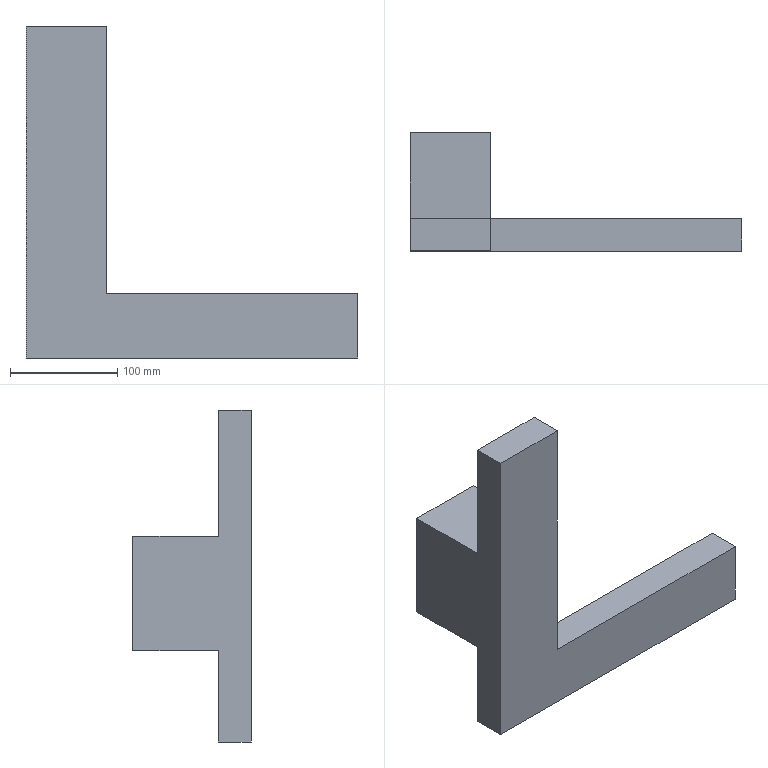Component | SolidWorks | MirrorPlate-2 | 1 solid | 19 faces | box 310 x 110.58 x 310 mm | volume 1628844 mm3 | plane 19
STEP:
#1=COLOUR_RGB('',0.7922,0.8196,0.9333);
#2=FILL_AREA_STYLE_COLOUR('',#1);
#3=FILL_AREA_STYLE('',(#2));
#4=SURFACE_STYLE_FILL_AREA(#3);
#5=SURFACE_SIDE_STYLE('',(#4));
#6=SURFACE_STYLE_USAGE(.BOTH.,#5);
#7=PRESENTATION_STYLE_ASSIGNMENT((#6));
#8=CARTESIAN_POINT('',(-6.62,1.886,11.6));
#9=VERTEX_POINT('',#8);
#10=CARTESIAN_POINT('',(-6.131,1.04,11.6));
#11=VERTEX_POINT('',#10);
#12=CARTESIAN_POINT('',(-6.131,1.04,11.6));
#13=DIRECTION('',(0.5,-0.866,-0.));
#14=VECTOR('',#13,39.37);
#15=LINE('',#12,#14);
#16=EDGE_CURVE('',#9,#11,#15,.T.);
#17=ORIENTED_EDGE('',*,*,#16,.F.);
#18=CARTESIAN_POINT('',(-6.62,1.886,7.781));
#19=VERTEX_POINT('',#18);
#20=CARTESIAN_POINT('',(-6.62,1.886,3.726));
#21=DIRECTION('',(0.,-0.,1.));
#22=VECTOR('',#21,39.37);
#23=LINE('',#20,#22);
#24=EDGE_CURVE('',#19,#9,#23,.T.);
#25=ORIENTED_EDGE('',*,*,#24,.F.);
#26=CARTESIAN_POINT('',(-6.131,1.04,7.781));
#27=VERTEX_POINT('',#26);
#28=CARTESIAN_POINT('',(-6.713,2.047,7.781));
#29=DIRECTION('',(-0.5,0.866,0.));
#30=VECTOR('',#29,39.37);
#31=LINE('',#28,#30);
#32=EDGE_CURVE('',#27,#19,#31,.T.);
#33=ORIENTED_EDGE('',*,*,#32,.F.);
#34=CARTESIAN_POINT('',(-6.131,1.04,3.726));
#35=DIRECTION('',(0.,-0.,1.));
#36=VECTOR('',#35,39.37);
#37=LINE('',#34,#36);
#38=EDGE_CURVE('',#27,#11,#37,.T.);
#39=ORIENTED_EDGE('',*,*,#38,.T.);
#40=EDGE_LOOP('',(#17,#25,#33,#39));
#41=FACE_OUTER_BOUND('',#40,.T.);
#42=CARTESIAN_POINT('',(-6.131,1.04,3.726));
#43=DIRECTION('',(0.866,0.5,0.));
#44=DIRECTION('',(0.5,-0.866,-0.));
#45=AXIS2_PLACEMENT_3D('',#42,#43,#44);
#46=PLANE('',#45);
#47=ADVANCED_FACE('',(#41),#46,.F.);
#48=CARTESIAN_POINT('',(-6.62,0.1934,11.6));
#49=VERTEX_POINT('',#48);
#50=CARTESIAN_POINT('',(-6.62,0.1934,11.6));
#51=DIRECTION('',(-0.5,-0.866,-0.));
#52=VECTOR('',#51,39.37);
#53=LINE('',#50,#52);
#54=EDGE_CURVE('',#11,#49,#53,.T.);
#55=ORIENTED_EDGE('',*,*,#54,.F.);
#56=ORIENTED_EDGE('',*,*,#38,.F.);
#57=CARTESIAN_POINT('',(-6.62,0.1934,7.781));
#58=VERTEX_POINT('',#57);
#59=CARTESIAN_POINT('',(-5.349,2.394,7.781));
#60=DIRECTION('',(0.5,0.866,0.));
#61=VECTOR('',#60,39.37);
#62=LINE('',#59,#61);
#63=EDGE_CURVE('',#58,#27,#62,.T.);
#64=ORIENTED_EDGE('',*,*,#63,.F.);
#65=CARTESIAN_POINT('',(-6.62,0.1934,3.726));
#66=DIRECTION('',(0.,-0.,1.));
#67=VECTOR('',#66,39.37);
#68=LINE('',#65,#67);
#69=EDGE_CURVE('',#58,#49,#68,.T.);
#70=ORIENTED_EDGE('',*,*,#69,.T.);
#71=EDGE_LOOP('',(#55,#56,#64,#70));
#72=FACE_OUTER_BOUND('',#71,.T.);
#73=CARTESIAN_POINT('',(-6.62,0.1934,3.726));
#74=DIRECTION('',(0.866,-0.5,-0.));
#75=DIRECTION('',(-0.5,-0.866,-0.));
#76=AXIS2_PLACEMENT_3D('',#73,#74,#75);
#77=PLANE('',#76);
#78=ADVANCED_FACE('',(#72),#77,.F.);
#79=CARTESIAN_POINT('',(-7.597,0.1934,11.6));
#80=VERTEX_POINT('',#79);
#81=CARTESIAN_POINT('',(-7.597,0.1934,11.6));
#82=DIRECTION('',(-1.,-0.,-0.));
#83=VECTOR('',#82,39.37);
#84=LINE('',#81,#83);
#85=EDGE_CURVE('',#49,#80,#84,.T.);
#86=ORIENTED_EDGE('',*,*,#85,.F.);
#87=ORIENTED_EDGE('',*,*,#69,.F.);
#88=CARTESIAN_POINT('',(-7.597,0.1934,7.781));
#89=VERTEX_POINT('',#88);
#90=CARTESIAN_POINT('',(-5.731,0.1934,7.781));
#91=DIRECTION('',(1.,0.,0.));
#92=VECTOR('',#91,39.37);
#93=LINE('',#90,#92);
#94=EDGE_CURVE('',#89,#58,#93,.T.);
#95=ORIENTED_EDGE('',*,*,#94,.F.);
#96=CARTESIAN_POINT('',(-7.597,0.1934,3.726));
#97=DIRECTION('',(0.,-0.,1.));
#98=VECTOR('',#97,39.37);
#99=LINE('',#96,#98);
#100=EDGE_CURVE('',#89,#80,#99,.T.);
#101=ORIENTED_EDGE('',*,*,#100,.T.);
#102=EDGE_LOOP('',(#86,#87,#95,#101));
#103=FACE_OUTER_BOUND('',#102,.T.);
#104=CARTESIAN_POINT('',(-7.597,0.1934,3.726));
#105=DIRECTION('',(0.,-1.,-0.));
#106=DIRECTION('',(-1.,-0.,-0.));
#107=AXIS2_PLACEMENT_3D('',#104,#105,#106);
#108=PLANE('',#107);
#109=ADVANCED_FACE('',(#103),#108,.F.);
#110=CARTESIAN_POINT('',(-8.086,1.04,11.6));
#111=VERTEX_POINT('',#110);
#112=CARTESIAN_POINT('',(-8.086,1.04,11.6));
#113=DIRECTION('',(-0.5,0.866,0.));
#114=VECTOR('',#113,39.37);
#115=LINE('',#112,#114);
#116=EDGE_CURVE('',#80,#111,#115,.T.);
#117=ORIENTED_EDGE('',*,*,#116,.F.);
#118=ORIENTED_EDGE('',*,*,#100,.F.);
#119=CARTESIAN_POINT('',(-8.086,1.04,7.781));
#120=VERTEX_POINT('',#119);
#121=CARTESIAN_POINT('',(-8.179,1.201,7.781));
#122=DIRECTION('',(0.5,-0.866,-0.));
#123=VECTOR('',#122,39.37);
#124=LINE('',#121,#123);
#125=EDGE_CURVE('',#120,#89,#124,.T.);
#126=ORIENTED_EDGE('',*,*,#125,.F.);
#127=CARTESIAN_POINT('',(-8.086,1.04,3.726));
#128=DIRECTION('',(0.,-0.,1.));
#129=VECTOR('',#128,39.37);
#130=LINE('',#127,#129);
#131=EDGE_CURVE('',#120,#111,#130,.T.);
#132=ORIENTED_EDGE('',*,*,#131,.T.);
#133=EDGE_LOOP('',(#117,#118,#126,#132));
#134=FACE_OUTER_BOUND('',#133,.T.);
#135=CARTESIAN_POINT('',(-8.086,1.04,3.726));
#136=DIRECTION('',(-0.866,-0.5,-0.));
#137=DIRECTION('',(-0.5,0.866,0.));
#138=AXIS2_PLACEMENT_3D('',#135,#136,#137);
#139=PLANE('',#138);
#140=ADVANCED_FACE('',(#134),#139,.F.);
#141=CARTESIAN_POINT('',(-7.597,1.886,11.6));
#142=VERTEX_POINT('',#141);
#143=CARTESIAN_POINT('',(-7.597,1.886,11.6));
#144=DIRECTION('',(0.5,0.866,0.));
#145=VECTOR('',#144,39.37);
#146=LINE('',#143,#145);
#147=EDGE_CURVE('',#111,#142,#146,.T.);
#148=ORIENTED_EDGE('',*,*,#147,.F.);
#149=ORIENTED_EDGE('',*,*,#131,.F.);
#150=CARTESIAN_POINT('',(-7.597,1.886,7.781));
#151=VERTEX_POINT('',#150);
#152=CARTESIAN_POINT('',(-6.815,3.241,7.781));
#153=DIRECTION('',(-0.5,-0.866,-0.));
#154=VECTOR('',#153,39.37);
#155=LINE('',#152,#154);
#156=EDGE_CURVE('',#151,#120,#155,.T.);
#157=ORIENTED_EDGE('',*,*,#156,.F.);
#158=CARTESIAN_POINT('',(-7.597,1.886,3.726));
#159=DIRECTION('',(0.,-0.,1.));
#160=VECTOR('',#159,39.37);
#161=LINE('',#158,#160);
#162=EDGE_CURVE('',#151,#142,#161,.T.);
#163=ORIENTED_EDGE('',*,*,#162,.T.);
#164=EDGE_LOOP('',(#148,#149,#157,#163));
#165=FACE_OUTER_BOUND('',#164,.T.);
#166=CARTESIAN_POINT('',(-7.597,1.886,3.726));
#167=DIRECTION('',(-0.866,0.5,0.));
#168=DIRECTION('',(0.5,0.866,0.));
#169=AXIS2_PLACEMENT_3D('',#166,#167,#168);
#170=PLANE('',#169);
#171=ADVANCED_FACE('',(#165),#170,.F.);
#172=CARTESIAN_POINT('',(-6.62,1.886,11.6));
#173=DIRECTION('',(1.,-0.,-0.));
#174=VECTOR('',#173,39.37);
#175=LINE('',#172,#174);
#176=EDGE_CURVE('',#142,#9,#175,.T.);
#177=ORIENTED_EDGE('',*,*,#176,.F.);
#178=ORIENTED_EDGE('',*,*,#162,.F.);
#179=CARTESIAN_POINT('',(-5.731,1.886,7.781));
#180=DIRECTION('',(-1.,0.,0.));
#181=VECTOR('',#180,39.37);
#182=LINE('',#179,#181);
#183=EDGE_CURVE('',#19,#151,#182,.T.);
#184=ORIENTED_EDGE('',*,*,#183,.F.);
#185=ORIENTED_EDGE('',*,*,#24,.T.);
#186=EDGE_LOOP('',(#177,#178,#184,#185));
#187=FACE_OUTER_BOUND('',#186,.T.);
#188=CARTESIAN_POINT('',(-6.62,1.886,3.726));
#189=DIRECTION('',(0.,1.,0.));
#190=DIRECTION('',(1.,-0.,-0.));
#191=AXIS2_PLACEMENT_3D('',#188,#189,#190);
#192=PLANE('',#191);
#193=ADVANCED_FACE('',(#187),#192,.F.);
#194=CARTESIAN_POINT('',(-5.731,-0.535,7.781));
#195=VERTEX_POINT('',#194);
#196=CARTESIAN_POINT('',(-8.683,-0.535,7.781));
#197=VERTEX_POINT('',#196);
#198=CARTESIAN_POINT('',(-5.731,-0.535,7.781));
#199=DIRECTION('',(-1.,0.,0.));
#200=VECTOR('',#199,39.37);
#201=LINE('',#198,#200);
#202=EDGE_CURVE('',#195,#197,#201,.T.);
#203=ORIENTED_EDGE('',*,*,#202,.F.);
#204=CARTESIAN_POINT('',(-5.731,-0.535,6.797));
#205=VERTEX_POINT('',#204);
#206=CARTESIAN_POINT('',(-5.731,-0.535,16.64));
#207=DIRECTION('',(0.,0.,-1.));
#208=VECTOR('',#207,39.37);
#209=LINE('',#206,#208);
#210=EDGE_CURVE('',#195,#205,#209,.T.);
#211=ORIENTED_EDGE('',*,*,#210,.T.);
#212=CARTESIAN_POINT('',(3.521,-0.535,6.797));
#213=VERTEX_POINT('',#212);
#214=CARTESIAN_POINT('',(-8.683,-0.535,6.797));
#215=DIRECTION('',(1.,-0.,-0.));
#216=VECTOR('',#215,39.37);
#217=LINE('',#214,#216);
#218=EDGE_CURVE('',#205,#213,#217,.T.);
#219=ORIENTED_EDGE('',*,*,#218,.T.);
#220=CARTESIAN_POINT('',(3.521,-0.535,4.435));
#221=VERTEX_POINT('',#220);
#222=CARTESIAN_POINT('',(3.521,-0.535,6.797));
#223=DIRECTION('',(0.,-0.,1.));
#224=VECTOR('',#223,39.37);
#225=LINE('',#222,#224);
#226=EDGE_CURVE('',#221,#213,#225,.T.);
#227=ORIENTED_EDGE('',*,*,#226,.F.);
#228=CARTESIAN_POINT('',(-8.683,-0.535,4.435));
#229=VERTEX_POINT('',#228);
#230=CARTESIAN_POINT('',(-8.683,-0.535,4.435));
#231=DIRECTION('',(1.,-0.,-0.));
#232=VECTOR('',#231,39.37);
#233=LINE('',#230,#232);
#234=EDGE_CURVE('',#229,#221,#233,.T.);
#235=ORIENTED_EDGE('',*,*,#234,.F.);
#236=CARTESIAN_POINT('',(-8.683,-0.535,6.797));
#237=DIRECTION('',(0.,-0.,1.));
#238=VECTOR('',#237,39.37);
#239=LINE('',#236,#238);
#240=EDGE_CURVE('',#229,#197,#239,.T.);
#241=ORIENTED_EDGE('',*,*,#240,.T.);
#242=EDGE_LOOP('',(#203,#211,#219,#227,#235,#241));
#243=FACE_OUTER_BOUND('',#242,.T.);
#244=CARTESIAN_POINT('',(-8.683,-0.535,6.797));
#245=DIRECTION('',(-0.,-1.,-0.));
#246=DIRECTION('',(1.,-0.,-0.));
#247=AXIS2_PLACEMENT_3D('',#244,#245,#246);
#248=PLANE('',#247);
#249=ADVANCED_FACE('',(#243),#248,.F.);
#250=CARTESIAN_POINT('',(-8.683,-0.535,11.994));
#251=VERTEX_POINT('',#250);
#252=CARTESIAN_POINT('',(-5.731,-0.535,11.994));
#253=VERTEX_POINT('',#252);
#254=CARTESIAN_POINT('',(-5.731,-0.535,11.994));
#255=DIRECTION('',(1.,-0.,-0.));
#256=VECTOR('',#255,39.37);
#257=LINE('',#254,#256);
#258=EDGE_CURVE('',#251,#253,#257,.T.);
#259=ORIENTED_EDGE('',*,*,#258,.F.);
#260=CARTESIAN_POINT('',(-8.683,-0.535,16.64));
#261=VERTEX_POINT('',#260);
#262=CARTESIAN_POINT('',(-8.683,-0.535,6.797));
#263=DIRECTION('',(0.,-0.,1.));
#264=VECTOR('',#263,39.37);
#265=LINE('',#262,#264);
#266=EDGE_CURVE('',#251,#261,#265,.T.);
#267=ORIENTED_EDGE('',*,*,#266,.T.);
#268=CARTESIAN_POINT('',(-5.731,-0.535,16.64));
#269=VERTEX_POINT('',#268);
#270=CARTESIAN_POINT('',(-5.731,-0.535,16.64));
#271=DIRECTION('',(1.,-0.,-0.));
#272=VECTOR('',#271,39.37);
#273=LINE('',#270,#272);
#274=EDGE_CURVE('',#261,#269,#273,.T.);
#275=ORIENTED_EDGE('',*,*,#274,.T.);
#276=CARTESIAN_POINT('',(-5.731,-0.535,16.64));
#277=DIRECTION('',(0.,0.,-1.));
#278=VECTOR('',#277,39.37);
#279=LINE('',#276,#278);
#280=EDGE_CURVE('',#269,#253,#279,.T.);
#281=ORIENTED_EDGE('',*,*,#280,.T.);
#282=EDGE_LOOP('',(#259,#267,#275,#281));
#283=FACE_OUTER_BOUND('',#282,.T.);
#284=CARTESIAN_POINT('',(-8.683,-0.535,6.797));
#285=DIRECTION('',(-0.,-1.,-0.));
#286=DIRECTION('',(1.,-0.,-0.));
#287=AXIS2_PLACEMENT_3D('',#284,#285,#286);
#288=PLANE('',#287);
#289=ADVANCED_FACE('',(#283),#288,.F.);
#290=CARTESIAN_POINT('',(-5.731,-1.739,6.797));
#291=VERTEX_POINT('',#290);
#292=CARTESIAN_POINT('',(-5.731,-0.535,6.797));
#293=DIRECTION('',(-0.,-1.,-0.));
#294=VECTOR('',#293,39.37);
#295=LINE('',#292,#294);
#296=EDGE_CURVE('',#205,#291,#295,.T.);
#297=ORIENTED_EDGE('',*,*,#296,.T.);
#298=CARTESIAN_POINT('',(3.521,-1.739,6.797));
#299=VERTEX_POINT('',#298);
#300=CARTESIAN_POINT('',(-8.683,-1.739,6.797));
#301=DIRECTION('',(1.,-0.,-0.));
#302=VECTOR('',#301,39.37);
#303=LINE('',#300,#302);
#304=EDGE_CURVE('',#291,#299,#303,.T.);
#305=ORIENTED_EDGE('',*,*,#304,.T.);
#306=CARTESIAN_POINT('',(3.521,-0.535,6.797));
#307=DIRECTION('',(-0.,-1.,-0.));
#308=VECTOR('',#307,39.37);
#309=LINE('',#306,#308);
#310=EDGE_CURVE('',#213,#299,#309,.T.);
#311=ORIENTED_EDGE('',*,*,#310,.F.);
#312=ORIENTED_EDGE('',*,*,#218,.F.);
#313=EDGE_LOOP('',(#297,#305,#311,#312));
#314=FACE_OUTER_BOUND('',#313,.T.);
#315=CARTESIAN_POINT('',(-8.683,-0.535,6.797));
#316=DIRECTION('',(0.,0.,-1.));
#317=DIRECTION('',(1.,-0.,-0.));
#318=AXIS2_PLACEMENT_3D('',#315,#316,#317);
#319=PLANE('',#318);
#320=ADVANCED_FACE('',(#314),#319,.F.);
#321=CARTESIAN_POINT('',(3.521,-1.739,4.435));
#322=VERTEX_POINT('',#321);
#323=CARTESIAN_POINT('',(3.521,-1.739,6.797));
#324=DIRECTION('',(0.,0.,-1.));
#325=VECTOR('',#324,39.37);
#326=LINE('',#323,#325);
#327=EDGE_CURVE('',#299,#322,#326,.T.);
#328=ORIENTED_EDGE('',*,*,#327,.F.);
#329=ORIENTED_EDGE('',*,*,#304,.F.);
#330=CARTESIAN_POINT('',(-5.731,-1.739,16.64));
#331=VERTEX_POINT('',#330);
#332=CARTESIAN_POINT('',(-5.731,-1.739,16.64));
#333=DIRECTION('',(0.,0.,-1.));
#334=VECTOR('',#333,39.37);
#335=LINE('',#332,#334);
#336=EDGE_CURVE('',#331,#291,#335,.T.);
#337=ORIENTED_EDGE('',*,*,#336,.F.);
#338=CARTESIAN_POINT('',(-8.683,-1.739,16.64));
#339=VERTEX_POINT('',#338);
#340=CARTESIAN_POINT('',(-5.731,-1.739,16.64));
#341=DIRECTION('',(-1.,0.,0.));
#342=VECTOR('',#341,39.37);
#343=LINE('',#340,#342);
#344=EDGE_CURVE('',#331,#339,#343,.T.);
#345=ORIENTED_EDGE('',*,*,#344,.T.);
#346=CARTESIAN_POINT('',(-8.683,-1.739,4.435));
#347=VERTEX_POINT('',#346);
#348=CARTESIAN_POINT('',(-8.683,-1.739,6.797));
#349=DIRECTION('',(0.,0.,-1.));
#350=VECTOR('',#349,39.37);
#351=LINE('',#348,#350);
#352=EDGE_CURVE('',#339,#347,#351,.T.);
#353=ORIENTED_EDGE('',*,*,#352,.T.);
#354=CARTESIAN_POINT('',(-8.683,-1.739,4.435));
#355=DIRECTION('',(1.,-0.,-0.));
#356=VECTOR('',#355,39.37);
#357=LINE('',#354,#356);
#358=EDGE_CURVE('',#347,#322,#357,.T.);
#359=ORIENTED_EDGE('',*,*,#358,.T.);
#360=EDGE_LOOP('',(#328,#329,#337,#345,#353,#359));
#361=FACE_OUTER_BOUND('',#360,.T.);
#362=CARTESIAN_POINT('',(-8.683,-1.739,6.797));
#363=DIRECTION('',(0.,1.,0.));
#364=DIRECTION('',(-1.,0.,0.));
#365=AXIS2_PLACEMENT_3D('',#362,#363,#364);
#366=PLANE('',#365);
#367=ADVANCED_FACE('',(#361),#366,.F.);
#368=CARTESIAN_POINT('',(3.521,-0.535,4.435));
#369=DIRECTION('',(0.,1.,0.));
#370=VECTOR('',#369,39.37);
#371=LINE('',#368,#370);
#372=EDGE_CURVE('',#322,#221,#371,.T.);
#373=ORIENTED_EDGE('',*,*,#372,.F.);
#374=ORIENTED_EDGE('',*,*,#358,.F.);
#375=CARTESIAN_POINT('',(-8.683,-0.535,4.435));
#376=DIRECTION('',(0.,1.,0.));
#377=VECTOR('',#376,39.37);
#378=LINE('',#375,#377);
#379=EDGE_CURVE('',#347,#229,#378,.T.);
#380=ORIENTED_EDGE('',*,*,#379,.T.);
#381=ORIENTED_EDGE('',*,*,#234,.T.);
#382=EDGE_LOOP('',(#373,#374,#380,#381));
#383=FACE_OUTER_BOUND('',#382,.T.);
#384=CARTESIAN_POINT('',(-8.683,-0.535,4.435));
#385=DIRECTION('',(0.,-0.,1.));
#386=DIRECTION('',(-1.,0.,0.));
#387=AXIS2_PLACEMENT_3D('',#384,#385,#386);
#388=PLANE('',#387);
#389=ADVANCED_FACE('',(#383),#388,.F.);
#390=ORIENTED_EDGE('',*,*,#266,.F.);
#391=CARTESIAN_POINT('',(-8.683,2.615,11.994));
#392=VERTEX_POINT('',#391);
#393=CARTESIAN_POINT('',(-8.683,2.615,11.994));
#394=DIRECTION('',(-0.,-1.,-0.));
#395=VECTOR('',#394,39.37);
#396=LINE('',#393,#395);
#397=EDGE_CURVE('',#392,#251,#396,.T.);
#398=ORIENTED_EDGE('',*,*,#397,.F.);
#399=CARTESIAN_POINT('',(-8.683,2.615,7.781));
#400=VERTEX_POINT('',#399);
#401=CARTESIAN_POINT('',(-8.683,2.615,7.781));
#402=DIRECTION('',(0.,-0.,1.));
#403=VECTOR('',#402,39.37);
#404=LINE('',#401,#403);
#405=EDGE_CURVE('',#400,#392,#404,.T.);
#406=ORIENTED_EDGE('',*,*,#405,.F.);
#407=CARTESIAN_POINT('',(-8.683,2.615,7.781));
#408=DIRECTION('',(-0.,-1.,-0.));
#409=VECTOR('',#408,39.37);
#410=LINE('',#407,#409);
#411=EDGE_CURVE('',#400,#197,#410,.T.);
#412=ORIENTED_EDGE('',*,*,#411,.T.);
#413=ORIENTED_EDGE('',*,*,#240,.F.);
#414=ORIENTED_EDGE('',*,*,#379,.F.);
#415=ORIENTED_EDGE('',*,*,#352,.F.);
#416=CARTESIAN_POINT('',(-8.683,-0.535,16.64));
#417=DIRECTION('',(0.,1.,0.));
#418=VECTOR('',#417,39.37);
#419=LINE('',#416,#418);
#420=EDGE_CURVE('',#339,#261,#419,.T.);
#421=ORIENTED_EDGE('',*,*,#420,.T.);
#422=EDGE_LOOP('',(#390,#398,#406,#412,#413,#414,#415,#421));
#423=FACE_OUTER_BOUND('',#422,.T.);
#424=CARTESIAN_POINT('',(-8.683,-0.,-0.1851));
#425=DIRECTION('',(-1.,0.,0.));
#426=DIRECTION('',(0.,0.,-1.));
#427=AXIS2_PLACEMENT_3D('',#424,#425,#426);
#428=PLANE('',#427);
#429=ADVANCED_FACE('',(#423),#428,.T.);
#430=ORIENTED_EDGE('',*,*,#310,.T.);
#431=ORIENTED_EDGE('',*,*,#327,.T.);
#432=ORIENTED_EDGE('',*,*,#372,.T.);
#433=ORIENTED_EDGE('',*,*,#226,.T.);
#434=EDGE_LOOP('',(#430,#431,#432,#433));
#435=FACE_OUTER_BOUND('',#434,.T.);
#436=CARTESIAN_POINT('',(3.521,-0.,-0.1851));
#437=DIRECTION('',(-1.,0.,0.));
#438=DIRECTION('',(0.,0.,-1.));
#439=AXIS2_PLACEMENT_3D('',#436,#437,#438);
#440=PLANE('',#439);
#441=ADVANCED_FACE('',(#435),#440,.F.);
#442=CARTESIAN_POINT('',(-5.731,2.615,11.994));
#443=VERTEX_POINT('',#442);
#444=CARTESIAN_POINT('',(-5.731,2.615,11.994));
#445=DIRECTION('',(-0.,-1.,-0.));
#446=VECTOR('',#445,39.37);
#447=LINE('',#444,#446);
#448=EDGE_CURVE('',#443,#253,#447,.T.);
#449=ORIENTED_EDGE('',*,*,#448,.T.);
#450=ORIENTED_EDGE('',*,*,#280,.F.);
#451=CARTESIAN_POINT('',(-5.731,-0.535,16.64));
#452=DIRECTION('',(-0.,-1.,-0.));
#453=VECTOR('',#452,39.37);
#454=LINE('',#451,#453);
#455=EDGE_CURVE('',#269,#331,#454,.T.);
#456=ORIENTED_EDGE('',*,*,#455,.T.);
#457=ORIENTED_EDGE('',*,*,#336,.T.);
#458=ORIENTED_EDGE('',*,*,#296,.F.);
#459=ORIENTED_EDGE('',*,*,#210,.F.);
#460=CARTESIAN_POINT('',(-5.731,2.615,7.781));
#461=VERTEX_POINT('',#460);
#462=CARTESIAN_POINT('',(-5.731,2.615,7.781));
#463=DIRECTION('',(-0.,-1.,-0.));
#464=VECTOR('',#463,39.37);
#465=LINE('',#462,#464);
#466=EDGE_CURVE('',#461,#195,#465,.T.);
#467=ORIENTED_EDGE('',*,*,#466,.F.);
#468=CARTESIAN_POINT('',(-5.731,2.615,7.781));
#469=DIRECTION('',(0.,0.,-1.));
#470=VECTOR('',#469,39.37);
#471=LINE('',#468,#470);
#472=EDGE_CURVE('',#443,#461,#471,.T.);
#473=ORIENTED_EDGE('',*,*,#472,.F.);
#474=EDGE_LOOP('',(#449,#450,#456,#457,#458,#459,#467,#473));
#475=FACE_OUTER_BOUND('',#474,.T.);
#476=CARTESIAN_POINT('',(-5.731,-0.535,16.64));
#477=DIRECTION('',(-1.,0.,0.));
#478=DIRECTION('',(0.,0.,-1.));
#479=AXIS2_PLACEMENT_3D('',#476,#477,#478);
#480=PLANE('',#479);
#481=ADVANCED_FACE('',(#475),#480,.F.);
#482=ORIENTED_EDGE('',*,*,#455,.F.);
#483=ORIENTED_EDGE('',*,*,#274,.F.);
#484=ORIENTED_EDGE('',*,*,#420,.F.);
#485=ORIENTED_EDGE('',*,*,#344,.F.);
#486=EDGE_LOOP('',(#482,#483,#484,#485));
#487=FACE_OUTER_BOUND('',#486,.T.);
#488=CARTESIAN_POINT('',(3.521,-0.,16.64));
#489=DIRECTION('',(0.,-0.,1.));
#490=DIRECTION('',(-1.,0.,0.));
#491=AXIS2_PLACEMENT_3D('',#488,#489,#490);
#492=PLANE('',#491);
#493=ADVANCED_FACE('',(#487),#492,.T.);
#494=ORIENTED_EDGE('',*,*,#63,.T.);
#495=ORIENTED_EDGE('',*,*,#32,.T.);
#496=ORIENTED_EDGE('',*,*,#183,.T.);
#497=ORIENTED_EDGE('',*,*,#156,.T.);
#498=ORIENTED_EDGE('',*,*,#125,.T.);
#499=ORIENTED_EDGE('',*,*,#94,.T.);
#500=EDGE_LOOP('',(#494,#495,#496,#497,#498,#499));
#501=FACE_BOUND('',#500,.T.);
#502=ORIENTED_EDGE('',*,*,#466,.T.);
#503=ORIENTED_EDGE('',*,*,#202,.T.);
#504=ORIENTED_EDGE('',*,*,#411,.F.);
#505=CARTESIAN_POINT('',(-5.731,2.615,7.781));
#506=DIRECTION('',(-1.,0.,0.));
#507=VECTOR('',#506,39.37);
#508=LINE('',#505,#507);
#509=EDGE_CURVE('',#461,#400,#508,.T.);
#510=ORIENTED_EDGE('',*,*,#509,.F.);
#511=EDGE_LOOP('',(#502,#503,#504,#510));
#512=FACE_OUTER_BOUND('',#511,.T.);
#513=CARTESIAN_POINT('',(-5.731,2.615,7.781));
#514=DIRECTION('',(0.,-0.,1.));
#515=DIRECTION('',(1.,-0.,-0.));
#516=AXIS2_PLACEMENT_3D('',#513,#514,#515);
#517=PLANE('',#516);
#518=ADVANCED_FACE('',(#501,#512),#517,.F.);
#519=ORIENTED_EDGE('',*,*,#397,.T.);
#520=ORIENTED_EDGE('',*,*,#258,.T.);
#521=ORIENTED_EDGE('',*,*,#448,.F.);
#522=CARTESIAN_POINT('',(-5.731,2.615,11.994));
#523=DIRECTION('',(1.,-0.,-0.));
#524=VECTOR('',#523,39.37);
#525=LINE('',#522,#524);
#526=EDGE_CURVE('',#392,#443,#525,.T.);
#527=ORIENTED_EDGE('',*,*,#526,.F.);
#528=EDGE_LOOP('',(#519,#520,#521,#527));
#529=FACE_OUTER_BOUND('',#528,.T.);
#530=CARTESIAN_POINT('',(-5.731,2.615,11.994));
#531=DIRECTION('',(0.,0.,-1.));
#532=DIRECTION('',(-1.,0.,0.));
#533=AXIS2_PLACEMENT_3D('',#530,#531,#532);
#534=PLANE('',#533);
#535=ADVANCED_FACE('',(#529),#534,.F.);
#536=ORIENTED_EDGE('',*,*,#472,.T.);
#537=ORIENTED_EDGE('',*,*,#509,.T.);
#538=ORIENTED_EDGE('',*,*,#405,.T.);
#539=ORIENTED_EDGE('',*,*,#526,.T.);
#540=EDGE_LOOP('',(#536,#537,#538,#539));
#541=FACE_OUTER_BOUND('',#540,.T.);
#542=CARTESIAN_POINT('',(3.521,2.615,-0.1851));
#543=DIRECTION('',(0.,1.,0.));
#544=DIRECTION('',(1.,-0.,-0.));
#545=AXIS2_PLACEMENT_3D('',#542,#543,#544);
#546=PLANE('',#545);
#547=ADVANCED_FACE('',(#541),#546,.T.);
#548=ORIENTED_EDGE('',*,*,#176,.T.);
#549=ORIENTED_EDGE('',*,*,#16,.T.);
#550=ORIENTED_EDGE('',*,*,#54,.T.);
#551=ORIENTED_EDGE('',*,*,#85,.T.);
#552=ORIENTED_EDGE('',*,*,#116,.T.);
#553=ORIENTED_EDGE('',*,*,#147,.T.);
#554=EDGE_LOOP('',(#548,#549,#550,#551,#552,#553));
#555=FACE_OUTER_BOUND('',#554,.T.);
#556=CARTESIAN_POINT('',(3.521,-0.,11.6));
#557=DIRECTION('',(0.,-0.,1.));
#558=DIRECTION('',(1.,-0.,-0.));
#559=AXIS2_PLACEMENT_3D('',#556,#557,#558);
#560=PLANE('',#559);
#561=ADVANCED_FACE('',(#555),#560,.F.);
#562=CLOSED_SHELL('',(#47,#78,#109,#140,#171,#193,#249,#289,#320,#367,#389,#429,#441,#481,#493,#518,#535,#547,#561));
#563=MANIFOLD_SOLID_BREP('',#562);
#564=STYLED_ITEM('',(#7),#563);
#565=(LENGTH_UNIT()NAMED_UNIT(*)SI_UNIT($,.METRE.));
#566=LENGTH_MEASURE_WITH_UNIT(LENGTH_MEASURE(0.0254),#565);
#567=DIMENSIONAL_EXPONENTS(1.,0.,0.,0.,0.,0.,0.);
#568=(CONVERSION_BASED_UNIT('',#566)LENGTH_UNIT()NAMED_UNIT(#567));
#569=UNCERTAINTY_MEASURE_WITH_UNIT(LENGTH_MEASURE(0.00001),#568,'','');
#570=(NAMED_UNIT(*)PLANE_ANGLE_UNIT()SI_UNIT($,.RADIAN.));
#571=(NAMED_UNIT(*)SI_UNIT($,.STERADIAN.)SOLID_ANGLE_UNIT());
#572=(GEOMETRIC_REPRESENTATION_CONTEXT(3)GLOBAL_UNCERTAINTY_ASSIGNED_CONTEXT((#569))GLOBAL_UNIT_ASSIGNED_CONTEXT((#568,#570,#571))REPRESENTATION_CONTEXT('',''));
#573=MECHANICAL_DESIGN_GEOMETRIC_PRESENTATION_REPRESENTATION('',(#564),#572);
#574=PRESENTATION_LAYER_ASSIGNMENT('','',(#564));
#575=CARTESIAN_POINT('',(0.,0.,0.));
#576=DIRECTION('',(0.,0.,1.));
#577=DIRECTION('',(1.,0.,0.));
#578=AXIS2_PLACEMENT_3D('',#575,#576,#577);
#579=(LENGTH_UNIT()NAMED_UNIT(*)SI_UNIT($,.METRE.));
#580=LENGTH_MEASURE_WITH_UNIT(LENGTH_MEASURE(0.0254),#579);
#581=DIMENSIONAL_EXPONENTS(1.,0.,0.,0.,0.,0.,0.);
#582=(CONVERSION_BASED_UNIT('',#580)LENGTH_UNIT()NAMED_UNIT(#581));
#583=UNCERTAINTY_MEASURE_WITH_UNIT(LENGTH_MEASURE(0.00001),#582,'','');
#584=(NAMED_UNIT(*)PLANE_ANGLE_UNIT()SI_UNIT($,.RADIAN.));
#585=(NAMED_UNIT(*)SI_UNIT($,.STERADIAN.)SOLID_ANGLE_UNIT());
#586=(GEOMETRIC_REPRESENTATION_CONTEXT(3)GLOBAL_UNCERTAINTY_ASSIGNED_CONTEXT((#583))GLOBAL_UNIT_ASSIGNED_CONTEXT((#582,#584,#585))REPRESENTATION_CONTEXT('',''));
#587=ADVANCED_BREP_SHAPE_REPRESENTATION('',(#563,#578),#586);